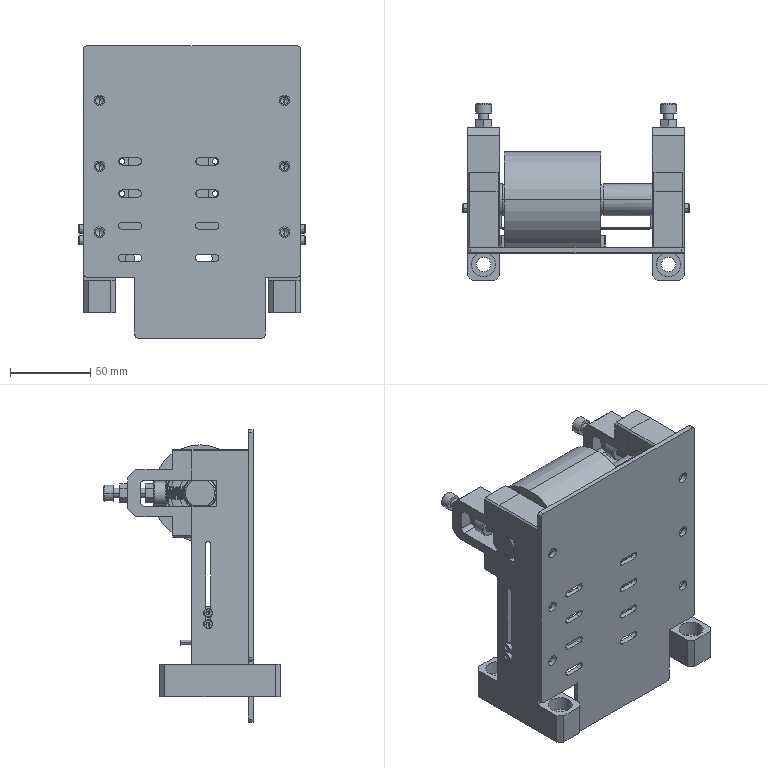Assembly | SolidWorks | mm | 29 component files | 29 solids | 735 faces | box 141 x 110 x 182 mm | volume 485433 mm3 | plane 358 | cylinder 253 | cone 104 | spline 20 | commonest cylinder face diameters 4.5 x24 5 x24 9 x24 6 x22 6.6 x20 15 x20 3.2 x18 4 x14
Bill of materials:
BAY6004ZZBearing | 2 |  | Thick annular ring with a central through bore, flat parallel end faces and slightly rounded edges; a faint concentric line on the end face between bore and outer edge.
B-TRD899MINI-2213-01FiberOpticBracket | 1 | SUS201 | Bent sheet bracket with a U-shaped profile: a long flat web with two 90-degree end flanges on the same side. The web has one long horizontal slot and one short slot at right angles to it. Each flange has two parallel elongated slots. Corners are rounded.
B-TRD899MINI-2213-02DesiccantBasePlate | 1 | SUS201 | Thin flat plate with a stepped outline: a wider rectangular main area and a narrower rectangular tab on one edge. It has six round through holes in two outer columns of three and eight short slots in two inner columns of four. Corners are slightly rounded.
FQ-10 | 1 |  | Stepped solid cylindrical pin with three coaxial diameters: a short larger collar at one end, a long main body, and a smaller reduced-diameter section at the other end.
J-TRD899MINI-2213-01DesiccantPressingSupportPlate | 2 | 6061 | Rectangular prismatic bar with a rectangular notch cut into one side near one end. It has a long narrow slot through a side face and three round holes along one narrow face, with chamfered or countersunk entries.
J-TRD899MINI-2213-02BracketVerticalPlate | 2 | 6061 | Rectangular block with chamfered vertical corners and four round through holes in a single row. In the isometric view the two outer holes look counterbored (a larger diameter with a step) and the two inner holes are plain.
J-TRD899MINI-2213-03PressingWheelSupport | 2 | 6061 | Prismatic block whose side profile is a hook or 'b' shape: a central closed C-shaped loop with rounded inner corners and chamfered outer corners, plus two offset rectangular lugs extending from the top and bottom. Round through holes pass through the lugs and the loop face.
J-TRD899MINI-2213-04PressingWheelAxis | 1 | 45 | Solid cylindrical shaft with flats machined at both ends, two narrow circumferential grooves along the body, and chamfered ends. The end sections look slightly reduced or flatted compared with the middle.
J-TRD899MINI-2213-05PressingWheel | 1 | Urethane | Plain cylindrical tube or sleeve with a uniform wall and a concentric through bore. Its length is roughly equal to its outer diameter, and the end faces are flat.
J-TRD899MINI-2213-06SpringAdjustmentWasher | 2 | 45 | Thick cylindrical spacer or ring with a central through bore and chamfered outer edges on both end faces. Its length is about half its outer diameter.
J-TRD899MINI-2213-07DesiccantSlot | 2 | 6061 | Rectangular block with a rabbet that gives an L-shaped cross section along one end, chamfered corners, and two round through holes on one face.
TAC21-M3-L30Screw | 4 |  | Headed pin: a short cylindrical head with chamfered edges and a long, slender, smooth cylindrical shank with a chamfered tip.
TAD01-M6-L30Screw | 2 |  | Headed cylindrical pin: a long, plain round shank with a short, larger-diameter cylindrical head at one end. Both ends have small chamfers.
TBK55-M6HexNut | 4 |  | Hexagonal nut-like block with a plain round hole through the centre and chamfered corners on at least one face.
YWF-D8-L25CompressionSpring | 2 |  | Helical coil of round wire with a constant coil diameter and even pitch. Both ends are cut off plainly, with no closed or flattened end coils.
Mates:
1. coincident | J-TRD899MINI-2213-02BracketVerticalPlate-1 face at (-16.663, 45.996, 85) dir (0, 1, 0) | J-TRD899MINI-2213-02BracketVerticalPlate-2 face at (-131.663, 45.996, 85) dir (0, 1, 0)
2. coincident | J-TRD899MINI-2213-02BracketVerticalPlate-1 face at (-6.663, 8.496, 85) dir (0, 0, 1) | J-TRD899MINI-2213-02BracketVerticalPlate-2 face at (-121.663, 8.496, 85) dir (0, 0, 1)
3. coincident | J-TRD899MINI-2213-02BracketVerticalPlate-1 face at (-6.663, 8.496, 85) dir (0, 0, 1) | J-TRD899MINI-2213-01DesiccantPressingSupportPlate-3 face at (3.337, -9.004, 85) dir (0, 0, -1)
4. concentric | J-TRD899MINI-2213-02BracketVerticalPlate-1 face at (-6.663, 17.496, 65) dir (0, 0, -1) r 7.5 | J-TRD899MINI-2213-01DesiccantPressingSupportPlate-3 face at (-6.663, 17.496, 85) dir (0, 0, -1) r 3.4
5. concentric | J-TRD899MINI-2213-02BracketVerticalPlate-1 face at (-6.663, -0.5041, 65) dir (0, 0, -1) r 7.5 | J-TRD899MINI-2213-01DesiccantPressingSupportPlate-3 face at (-6.663, -0.5041, 85) dir (0, 0, -1) r 3.4
6. coincident | J-TRD899MINI-2213-02BracketVerticalPlate-2 face at (-121.663, 8.496, 85) dir (0, 0, 1) | J-TRD899MINI-2213-01DesiccantPressingSupportPlate-4 face at (-111.663, -9.004, 85) dir (0, 0, -1)
7. concentric | J-TRD899MINI-2213-02BracketVerticalPlate-2 face at (-121.663, 17.496, 65) dir (0, 0, -1) r 7.5 | J-TRD899MINI-2213-01DesiccantPressingSupportPlate-4 face at (-121.663, 17.496, 85) dir (0, 0, -1) r 3.4
8. concentric | J-TRD899MINI-2213-02BracketVerticalPlate-2 face at (-121.663, -0.5041, 65) dir (0, 0, -1) r 7.5 | J-TRD899MINI-2213-01DesiccantPressingSupportPlate-4 face at (-121.663, -0.5041, 85) dir (0, 0, -1) r 3.4
9. coincident | J-TRD899MINI-2213-01DesiccantPressingSupportPlate-3 face at (-16.663, 8.496, 152) dir (-1, 0, 0) | B-TRD899MINI-2213-01FiberOpticBracket-1 face at (-16.663, 3.996, 106) dir (1, 0, 0)
10. distance | J-TRD899MINI-2213-02BracketVerticalPlate-2 face at (-111.663, -29.004, 85) dir (1, 0, 0) | J-TRD899MINI-2213-02BracketVerticalPlate-1 face at (-16.663, -29.004, 85) dir (-1, 0, 0)
11. concentric | J-TRD899MINI-2213-01DesiccantPressingSupportPlate-3 face at (-16.663, 15.996, 110) dir (1, 0, 0) r 1.6 | B-TRD899MINI-2213-01FiberOpticBracket-1 face at (-111.663, 15.996, 110) dir (1, 0, 0) r 1.6
12. parallel | J-TRD899MINI-2213-01DesiccantPressingSupportPlate-3 face at (3.337, 25.996, 219) dir (0, 1, 0) | B-TRD899MINI-2213-01FiberOpticBracket-1 face at (-16.663, 18.996, 121) dir (0, 1, 0)
13. coincident | B-TRD899MINI-2213-01FiberOpticBracket-1 face at (-64.163, 2.996, 106) dir (0, -1, 0) | FQ-10-1 face at (-102.663, 2.996, 98.5) dir (0, 1, 0)
14. concentric | B-TRD899MINI-2213-01FiberOpticBracket-1 face at (-102.663, 2.996, 98.5) dir (0, 1, 0) r 3.1 | FQ-10-1 face at (-102.663, 2.996, 98.5) dir (0, -1, 0) r 3
15. coincident | J-TRD899MINI-2213-01DesiccantPressingSupportPlate-3 face at (3.337, -9.004, 219) dir (0, -1, 0) | B-TRD899MINI-2213-02DesiccantBasePlate-1 face at (-64.163, -9.004, 140) dir (0, 1, 0)
16. concentric | J-TRD899MINI-2213-01DesiccantPressingSupportPlate-3 face at (-6.663, -9.004, 115) dir (0, -1, 0) r 2.5 | B-TRD899MINI-2213-02DesiccantBasePlate-1 face at (-6.663, -12.004, 115) dir (0, -1, 0) r 3.3
17. coincident | J-TRD899MINI-2213-01DesiccantPressingSupportPlate-3 face at (3.337, 8.496, 152) dir (1, 0, 0) | B-TRD899MINI-2213-02DesiccantBasePlate-1 face at (3.337, -12.004, 231) dir (1, 0, 0)
18. coincident | J-TRD899MINI-2213-01DesiccantPressingSupportPlate-4 face at (-111.663, 25.996, 219) dir (0, 1, 0) | J-TRD899MINI-2213-03PressingWheelSupport-1 face at (-111.663, 25.996, 164) dir (0, -1, 0)
19. coincident | J-TRD899MINI-2213-01DesiccantPressingSupportPlate-3 face at (3.337, 25.996, 219) dir (0, 1, 0) | J-TRD899MINI-2213-03PressingWheelSupport-2 face at (3.337, 25.996, 164) dir (0, -1, 0)
20. concentric | J-TRD899MINI-2213-01DesiccantPressingSupportPlate-4 face at (-121.663, 25.996, 213) dir (0, 1, 0) r 2.5 | J-TRD899MINI-2213-03PressingWheelSupport-1 face at (-121.663, 65.996, 213) dir (0, 1, 0) r 3.3
21. coincident | J-TRD899MINI-2213-01DesiccantPressingSupportPlate-4 face at (-131.663, 8.496, 152) dir (-1, 0, 0) | J-TRD899MINI-2213-03PressingWheelSupport-1 face at (-131.663, 45.996, 191.5) dir (-1, 0, 0)
22. concentric | J-TRD899MINI-2213-01DesiccantPressingSupportPlate-3 face at (-6.663, 25.996, 213) dir (0, 1, 0) r 2.5 | J-TRD899MINI-2213-03PressingWheelSupport-2 face at (-6.663, 65.996, 213) dir (0, 1, 0) r 3.3
23. coincident | J-TRD899MINI-2213-01DesiccantPressingSupportPlate-3 face at (3.337, 8.496, 152) dir (1, 0, 0) | J-TRD899MINI-2213-03PressingWheelSupport-2 face at (3.337, 45.996, 191.5) dir (1, 0, 0)
24. coincident | J-TRD899MINI-2213-03PressingWheelSupport-1 face at (-131.663, 45.996, 191.5) dir (-1, 0, 0) | J-TRD899MINI-2213-04PressingWheelAxis-1 face at (-131.663, 30.996, 191.6) dir (-1, 0, 0)
25. coincident | J-TRD899MINI-2213-03PressingWheelSupport-1 face at (-131.663, 55.496, 199.6) dir (0, 0, -1) | J-TRD899MINI-2213-04PressingWheelAxis-1 face at (-131.663, 10.996, 199.6) dir (0, 0, 1)
26. tangent | J-TRD899MINI-2213-04PressingWheelAxis-1 face at (3.337, 20.996, 191.6) dir (1, 0, 0) r 10 | J-TRD899MINI-2213-01DesiccantPressingSupportPlate-4 face at (-131.663, 10.996, 199.6) dir (0, 1, 0)
27. concentric | J-TRD899MINI-2213-04PressingWheelAxis-1 face at (3.337, 20.996, 191.6) dir (1, 0, 0) r 10 | J-TRD899MINI-2213-05PressingWheel-1 face at (-108.663, 20.996, 191.6) dir (-1, 0, 0) r 30
28. coincident | J-TRD899MINI-2213-04PressingWheelAxis-1 face at (-108.663, 30.996, 191.6) dir (-1, 0, 0) | J-TRD899MINI-2213-05PressingWheel-1 face at (-108.663, 50.996, 191.6) dir (-1, 0, 0)
29. coincident | J-TRD899MINI-2213-05PressingWheel-1 face at (-108.663, 50.996, 191.6) dir (-1, 0, 0) | BAY6004ZZBearing-1 face at (-108.663, 41.396, 191.6) dir (-1, 0, 0)
30. concentric | J-TRD899MINI-2213-05PressingWheel-1 face at (-108.663, 20.996, 191.6) dir (-1, 0, 0) r 30 | BAY6004ZZBearing-1 face at (-96.663, 20.996, 191.6) dir (-1, 0, 0) r 21
31. coincident | J-TRD899MINI-2213-05PressingWheel-1 face at (-48.663, 50.996, 191.6) dir (1, 0, 0) | BAY6004ZZBearing-2 face at (-48.663, 39.396, 191.6) dir (1, 0, 0)
32. concentric | J-TRD899MINI-2213-05PressingWheel-1 face at (-108.663, 20.996, 191.6) dir (-1, 0, 0) r 30 | BAY6004ZZBearing-2 face at (-48.663, 20.996, 191.6) dir (-1, 0, 0) r 21
33. coincident | J-TRD899MINI-2213-06SpringAdjustmentWasher-3 face at (-121.663, 49.996, 191.5) dir (0, 1, 0) | J-TRD899MINI-2213-06SpringAdjustmentWasher-4 face at (-6.663, 49.996, 191.5) dir (0, 1, 0)
34. distance | J-TRD899MINI-2213-06SpringAdjustmentWasher-4 face at (-6.663, 49.996, 191.5) dir (0, 1, 0) | J-TRD899MINI-2213-03PressingWheelSupport-2 face at (-16.663, 57.996, 185.9) dir (0, -1, 0)
35. concentric | J-TRD899MINI-2213-03PressingWheelSupport-2 face at (-6.663, 65.996, 191.5) dir (0, 1, 0) r 3 | J-TRD899MINI-2213-06SpringAdjustmentWasher-4 face at (-6.663, 49.996, 191.5) dir (0, 1, 0) r 3
36. concentric | J-TRD899MINI-2213-03PressingWheelSupport-1 face at (-121.663, 65.996, 191.5) dir (0, 1, 0) r 3 | J-TRD899MINI-2213-06SpringAdjustmentWasher-3 face at (-121.663, 49.996, 191.5) dir (0, 1, 0) r 3
37. concentric | J-TRD899MINI-2213-07DesiccantSlot-2 face at (-107.663, -1.004, 159) dir (0, 1, 0) r 1.65 | B-TRD899MINI-2213-02DesiccantBasePlate-1 face at (-107.663, -12.004, 159) dir (0, 1, 0) r 2.25
38. parallel | J-TRD899MINI-2213-01DesiccantPressingSupportPlate-4 face at (-111.663, 8.496, 152) dir (1, 0, 0) | J-TRD899MINI-2213-07DesiccantSlot-2 face at (-95.663, -4.004, 169) dir (1, 0, 0)
39. concentric | J-TRD899MINI-2213-07DesiccantSlot-1 face at (-49.663, -1.004, 159) dir (0, 1, 0) r 1.65 | B-TRD899MINI-2213-02DesiccantBasePlate-1 face at (-49.663, -12.004, 159) dir (0, 1, 0) r 2.25
40. parallel | J-TRD899MINI-2213-07DesiccantSlot-1 face at (-61.663, -4.004, 129) dir (-1, 0, 0) | J-TRD899MINI-2213-01DesiccantPressingSupportPlate-3 face at (-16.663, 8.496, 152) dir (-1, 0, 0)
41. coincident | YWF-D8-L25CompressionSpring-1 face at (-2.663, 44.995, 187.294) dir (0, 1, 0) | YWF-D8-L25CompressionSpring-2 face at (-117.663, 44.995, 187.294) dir (0, 1, 0)
42. coincident | J-TRD899MINI-2213-04PressingWheelAxis-1 face at (-6.663, 27.996, 191.6) dir (0, 1, 0) | YWF-D8-L25CompressionSpring-2 face at (-125.663, 27.996, 187.294) dir (0, -1, 0)
43. concentric | J-TRD899MINI-2213-06SpringAdjustmentWasher-4 face at (-6.663, 49.996, 191.5) dir (0, 1, 0) r 7.5 | YWF-D8-L25CompressionSpring-1 axis at (-6.663, 46.615, 191.5) dir (0, -1, 0)
44. concentric | J-TRD899MINI-2213-06SpringAdjustmentWasher-3 face at (-121.663, 49.996, 191.5) dir (0, 1, 0) r 7.5 | YWF-D8-L25CompressionSpring-2 axis at (-121.663, 46.615, 191.5) dir (0, -1, 0)
45. coincident | TAD01-M6-L30Screw-1 face at (-121.663, 80.996, 191.5) dir (0, 1, 0) | TAD01-M6-L30Screw-2 face at (-6.663, 80.996, 191.5) dir (0, 1, 0)
46. coincident | J-TRD899MINI-2213-06SpringAdjustmentWasher-4 face at (-2.163, 44.996, 191.5) dir (0, -1, 0) | TAD01-M6-L30Screw-1 face at (-121.663, 44.996, 189.113) dir (0, -1, 0)
47. concentric | J-TRD899MINI-2213-03PressingWheelSupport-1 face at (-121.663, 65.996, 191.5) dir (0, 1, 0) r 3 | TAD01-M6-L30Screw-1 face at (-121.663, 44.996, 191.5) dir (0, 1, 0) r 3
48. concentric | J-TRD899MINI-2213-03PressingWheelSupport-2 face at (-6.663, 65.996, 191.5) dir (0, 1, 0) r 3 | TAD01-M6-L30Screw-2 face at (-6.663, 44.996, 191.5) dir (0, 1, 0) r 3
49. coincident | J-TRD899MINI-2213-06SpringAdjustmentWasher-3 face at (-121.663, 49.996, 191.5) dir (0, 1, 0) | TBK55-M6HexNut-1 face at (-121.663, 49.996, 191.5) dir (0, -1, 0)
50. coincident | J-TRD899MINI-2213-03PressingWheelSupport-1 face at (-111.663, 65.996, 164) dir (0, 1, 0) | TBK55-M6HexNut-2 face at (-121.663, 65.996, 191.5) dir (0, -1, 0)
51. coincident | J-TRD899MINI-2213-06SpringAdjustmentWasher-4 face at (-6.663, 49.996, 191.5) dir (0, 1, 0) | TBK55-M6HexNut-3 face at (-6.663, 49.996, 191.5) dir (0, -1, 0)
52. coincident | J-TRD899MINI-2213-03PressingWheelSupport-2 face at (3.337, 65.996, 164) dir (0, 1, 0) | TBK55-M6HexNut-4 face at (-6.663, 65.996, 191.5) dir (0, -1, 0)
53. coincident | TAC21-M3-L30Screw-1 face at (-134.663, 15.996, 117) dir (-1, 0, 0) | TAC21-M3-L30Screw-2 face at (-134.663, 15.996, 110) dir (-1, 0, 0)
54. coincident | J-TRD899MINI-2213-01DesiccantPressingSupportPlate-4 face at (-131.663, 8.496, 152) dir (-1, 0, 0) | TAC21-M3-L30Screw-2 face at (-131.663, 18.746, 110) dir (1, 0, 0)
55. concentric | B-TRD899MINI-2213-01FiberOpticBracket-1 face at (-111.663, 15.996, 110) dir (1, 0, 0) r 1.6 | TAC21-M3-L30Screw-2 face at (-101.663, 15.996, 110) dir (-1, 0, 0) r 1.5
56. concentric | B-TRD899MINI-2213-01FiberOpticBracket-1 face at (-111.663, 15.996, 117) dir (1, 0, 0) r 1.6 | TAC21-M3-L30Screw-1 face at (-101.663, 15.996, 117) dir (-1, 0, 0) r 1.5
57. coincident | TAC21-M3-L30Screw-3 face at (6.337, 15.996, 117) dir (1, 0, 0) | TAC21-M3-L30Screw-4 face at (6.337, 15.996, 110) dir (1, 0, 0)
58. coincident | J-TRD899MINI-2213-01DesiccantPressingSupportPlate-3 face at (3.337, 8.496, 152) dir (1, 0, 0) | TAC21-M3-L30Screw-4 face at (3.337, 18.746, 110) dir (-1, 0, 0)
59. concentric | B-TRD899MINI-2213-01FiberOpticBracket-1 face at (-111.663, 15.996, 110) dir (1, 0, 0) r 1.6 | TAC21-M3-L30Screw-4 face at (-26.663, 15.996, 110) dir (1, 0, 0) r 1.5
60. concentric | B-TRD899MINI-2213-01FiberOpticBracket-1 face at (-111.663, 15.996, 117) dir (1, 0, 0) r 1.6 | TAC21-M3-L30Screw-3 face at (-26.663, 15.996, 117) dir (1, 0, 0) r 1.5
61. coincident | B-TRD899MINI-2213-02DesiccantBasePlate-1 face at (-64.163, -9.004, 140) dir (0, 1, 0) | J-TRD899MINI-2213-07DesiccantSlot-2 face at (-111.663, -9.004, 169) dir (0, -1, 0)
62. coincident | B-TRD899MINI-2213-02DesiccantBasePlate-1 face at (-64.163, -9.004, 140) dir (0, 1, 0) | J-TRD899MINI-2213-07DesiccantSlot-1 face at (-45.663, -9.004, 129) dir (0, -1, 0)
63. concentric | TAD01-M6-L30Screw-1 face at (-121.663, 44.996, 191.5) dir (0, 1, 0) r 3 | TBK55-M6HexNut-1 face at (-121.663, 49.996, 191.5) dir (0, 1, 0) r 3
64. concentric | TAD01-M6-L30Screw-1 face at (-121.663, 44.996, 191.5) dir (0, 1, 0) r 3 | TBK55-M6HexNut-2 face at (-121.663, 65.996, 191.5) dir (0, 1, 0) r 3
65. concentric | TAD01-M6-L30Screw-2 face at (-6.663, 44.996, 191.5) dir (0, 1, 0) r 3 | TBK55-M6HexNut-3 face at (-6.663, 49.996, 191.5) dir (0, 1, 0) r 3
66. concentric | TAD01-M6-L30Screw-2 face at (-6.663, 44.996, 191.5) dir (0, 1, 0) r 3 | TBK55-M6HexNut-4 face at (-6.663, 65.996, 191.5) dir (0, 1, 0) r 3